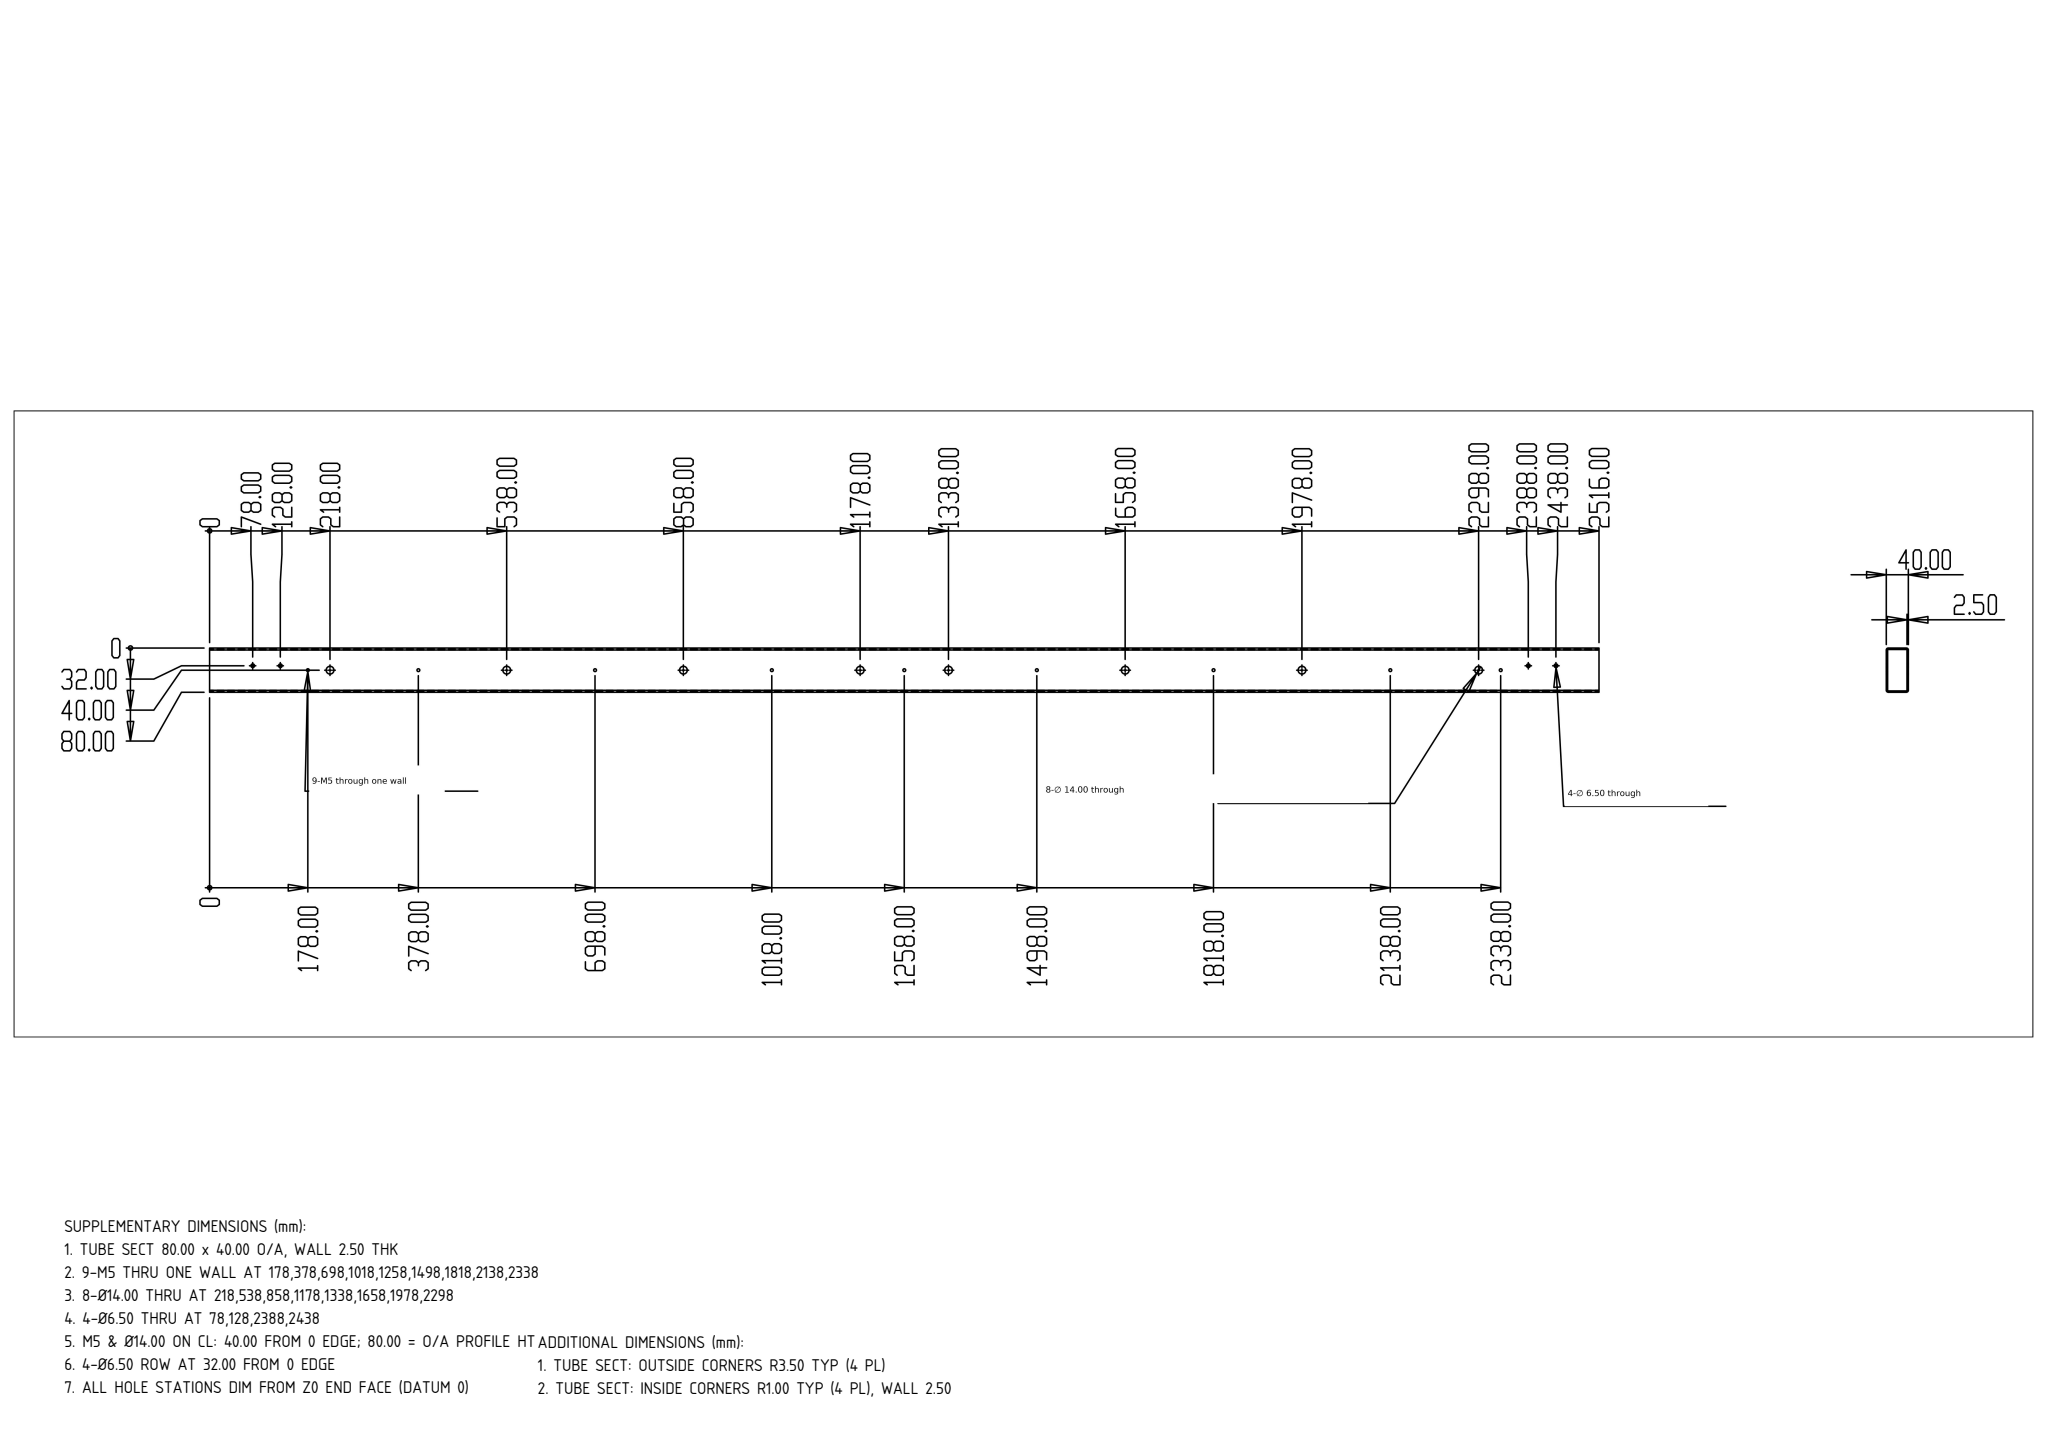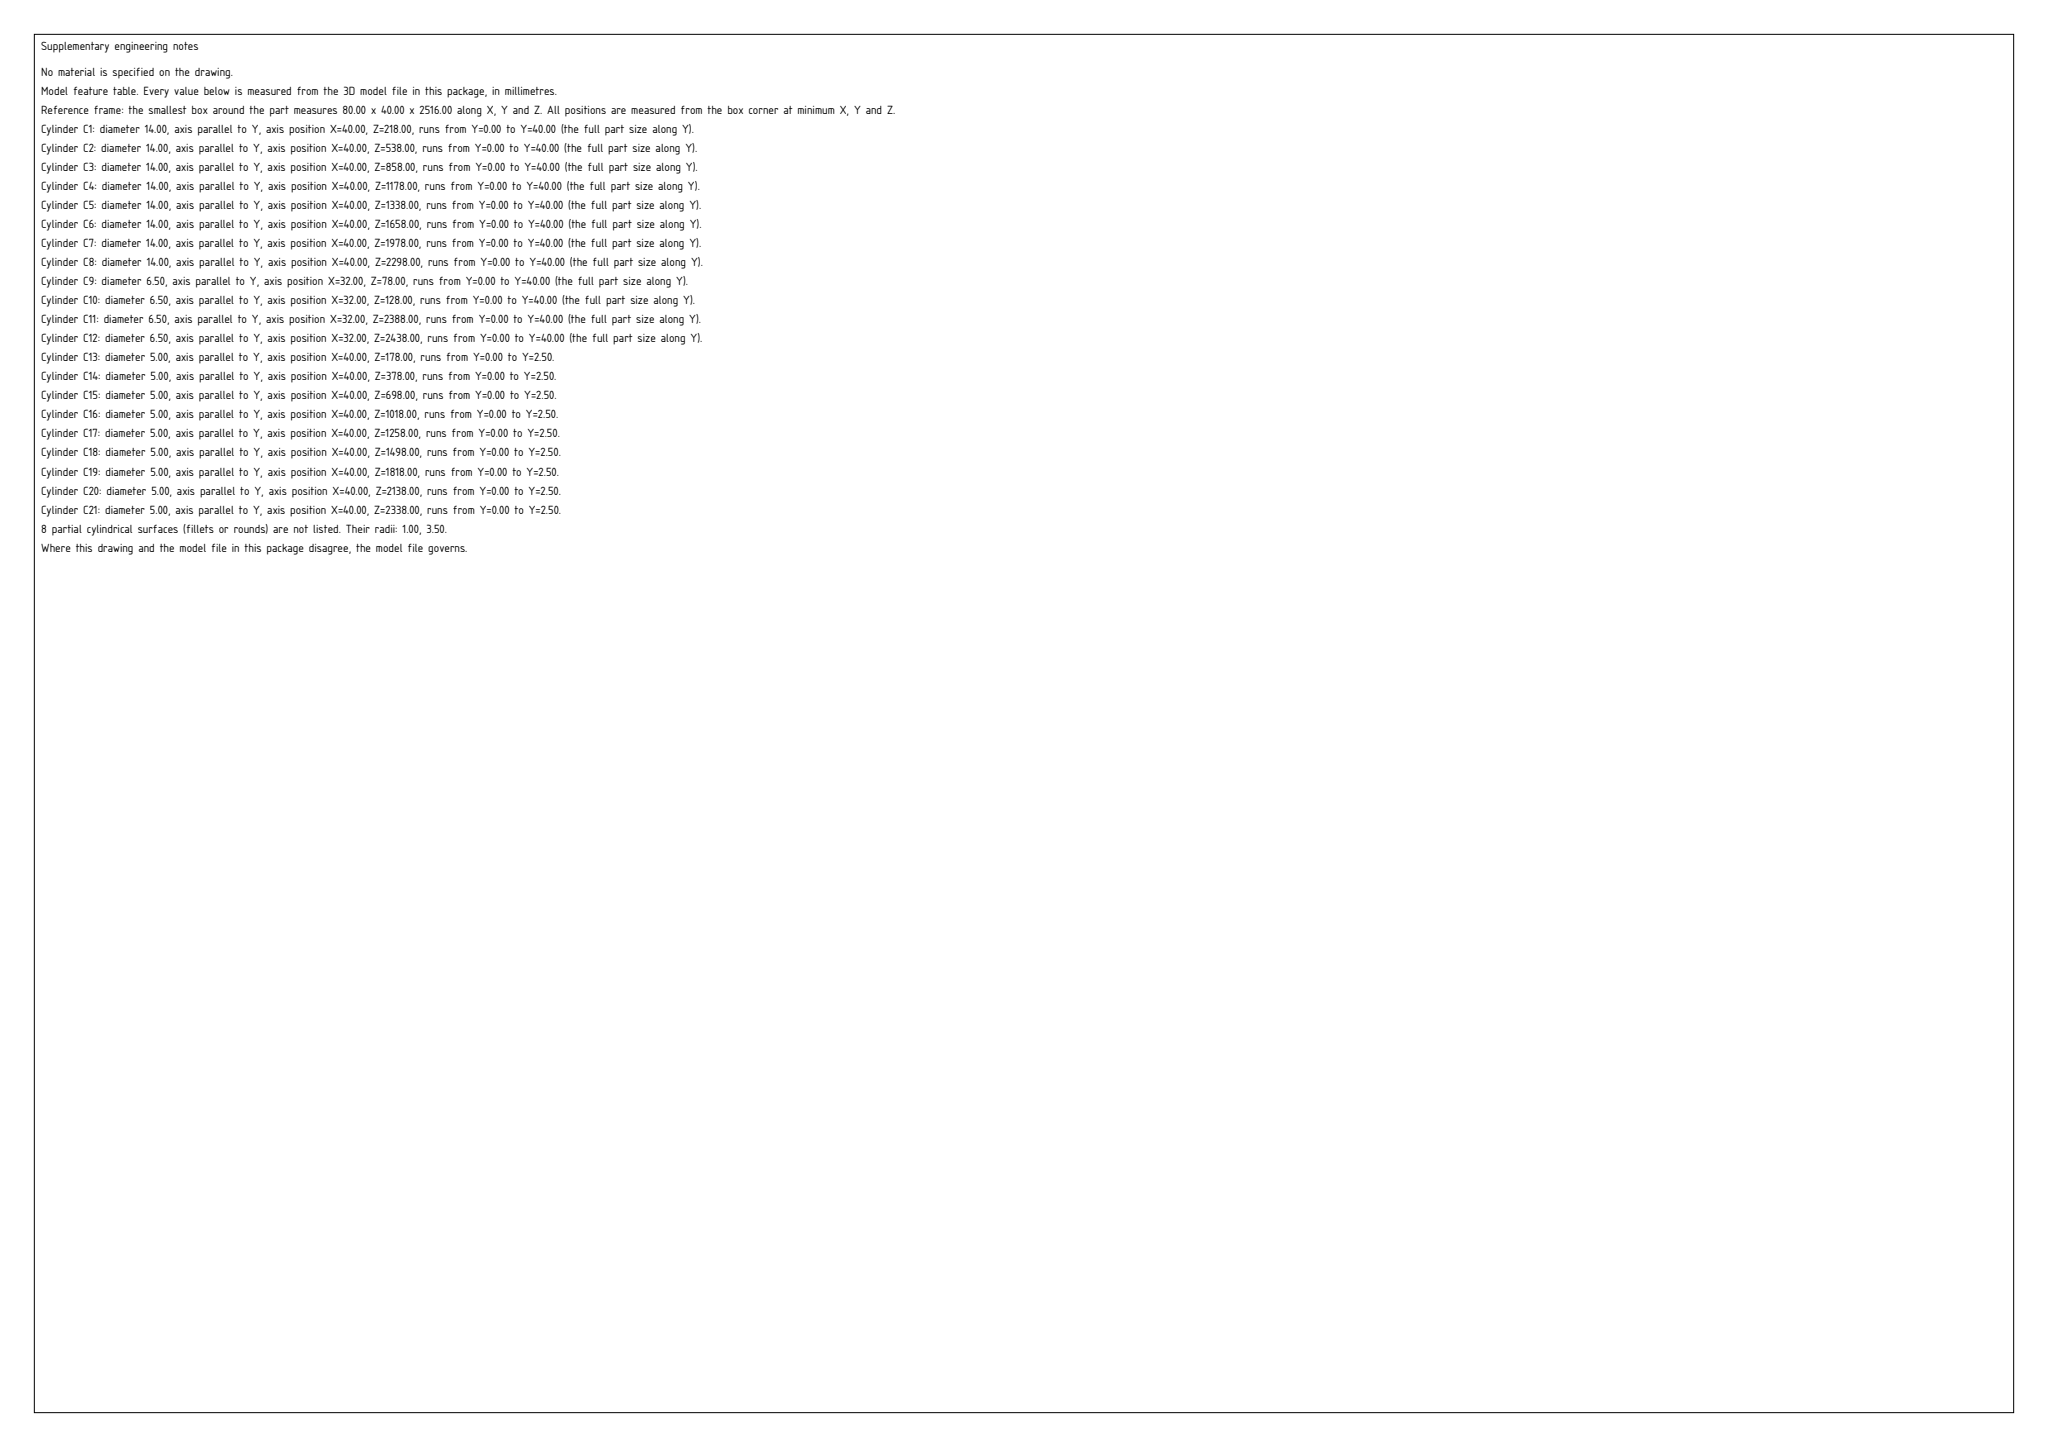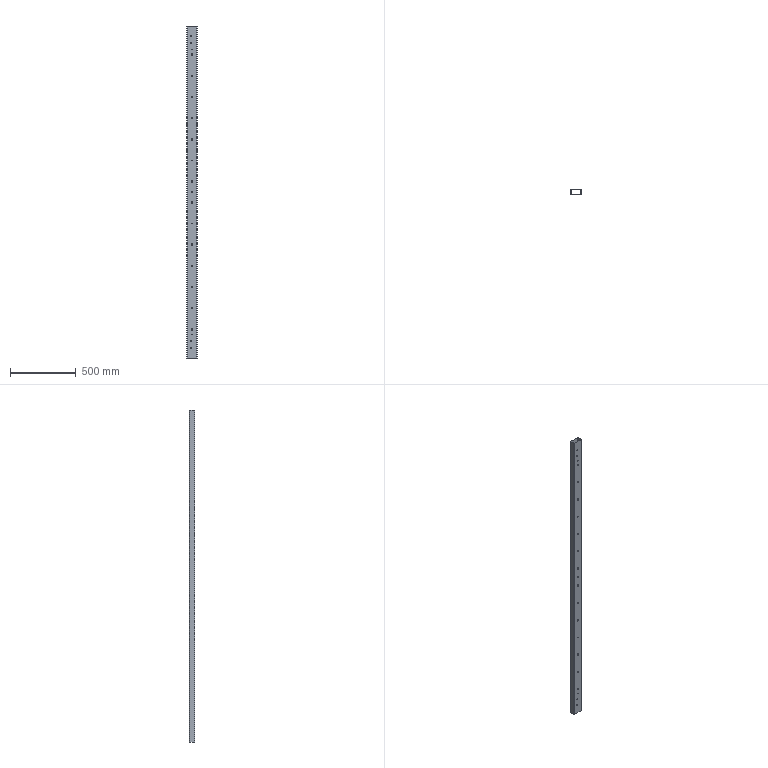Part | SolidWorks | mm | 1 solid | 84 faces | box 80 x 40 x 2516 mm | volume 1415140 mm3 | cylinder 74 | plane 10 | commonest cylinder face diameters 14 x32 5 x18 6.5 x16 7 x4 2 x4
build123d program:
from build123d import *

# Parameters (mm, degrees)
BOSS_EXTRUDE1_DEPTH = 2516
CUT_EXTRUDE1_REACH  = 2518.636
CUT_EXTRUDE2_START  = -37.5
CUT_EXTRUDE2_DEPTH  = 37.5


with BuildPart() as part:
    # Sketch1 → Boss-Extrude1 (new body)
    with BuildSketch(Plane.XY):
        with BuildLine():
            Line((40, -16.5), (40, 16.5))
            ThreePointArc((40, 16.5), (38.975, 18.975), (36.5, 20))
            Line((36.5, 20), (-36.5, 20))
            ThreePointArc((-36.5, 20), (-38.975, 18.975), (-40, 16.5))
            Line((-40, 16.5), (-40, -16.5))
            ThreePointArc((-40, -16.5), (-38.975, -18.975), (-36.5, -20))
            Line((-36.5, -20), (36.5, -20))
            ThreePointArc((36.5, -20), (38.975, -18.975), (40, -16.5))
        make_face()
        with BuildLine():
            Line((37.5, -16.5), (37.5, 16.5))
            ThreePointArc((37.5, 16.5), (37.207, 17.207), (36.5, 17.5))
            Line((36.5, 17.5), (-36.5, 17.5))
            ThreePointArc((-36.5, 17.5), (-37.207, 17.207), (-37.5, 16.5))
            Line((-37.5, 16.5), (-37.5, -16.5))
            ThreePointArc((-37.5, -16.5), (-37.207, -17.207), (-36.5, -17.5))
            Line((-36.5, -17.5), (36.5, -17.5))
            ThreePointArc((36.5, -17.5), (37.207, -17.207), (37.5, -16.5))
        make_face(mode=Mode.SUBTRACT)
    extrude(amount=BOSS_EXTRUDE1_DEPTH)

    # Cut-Extrude1: up to this face of the body (flat: up to its plane)
    cut_extrude1_end = Plane(part.part.faces().sort_by_distance((0, -20, 1258))[0])
    # Sketch2 → Cut-Extrude1 (cut, up to the picked face)
    with BuildSketch(Plane(origin=(0, 20, 0), x_dir=(1, 0, 0), z_dir=(0, 1, 0)), mode=Mode.PRIVATE) as cut_extrude1_sk1:
        with BuildLine():
            ThreePointArc((7, -2298), (0, -2291), (-7, -2298))
            ThreePointArc((-7, -2298), (0, -2305), (7, -2298))
        make_face()
    cut_extrude1_tool1 = split(extrude(cut_extrude1_sk1.sketch, amount=-CUT_EXTRUDE1_REACH, mode=Mode.PRIVATE), bisect_by=cut_extrude1_end, keep=Keep.BOTH, mode=Mode.PRIVATE)
    # Sketch2 → Cut-Extrude1 (cut, up to the picked face)
    with BuildSketch(Plane(origin=(0, 20, 0), x_dir=(1, 0, 0), z_dir=(0, 1, 0)), mode=Mode.PRIVATE) as cut_extrude1_sk2:
        with BuildLine():
            ThreePointArc((7, -218), (0, -211), (-7, -218))
            ThreePointArc((-7, -218), (0, -225), (7, -218))
        make_face()
    cut_extrude1_tool2 = split(extrude(cut_extrude1_sk2.sketch, amount=-CUT_EXTRUDE1_REACH, mode=Mode.PRIVATE), bisect_by=cut_extrude1_end, keep=Keep.BOTH, mode=Mode.PRIVATE)
    # Sketch2 → Cut-Extrude1 (cut, up to the picked face)
    with BuildSketch(Plane(origin=(0, 20, 0), x_dir=(1, 0, 0), z_dir=(0, 1, 0)), mode=Mode.PRIVATE) as cut_extrude1_sk3:
        with BuildLine():
            ThreePointArc((7, -1658), (0, -1651), (-7, -1658))
            ThreePointArc((-7, -1658), (0, -1665), (7, -1658))
        make_face()
    cut_extrude1_tool3 = split(extrude(cut_extrude1_sk3.sketch, amount=-CUT_EXTRUDE1_REACH, mode=Mode.PRIVATE), bisect_by=cut_extrude1_end, keep=Keep.BOTH, mode=Mode.PRIVATE)
    # Sketch2 → Cut-Extrude1 (cut, up to the picked face)
    with BuildSketch(Plane(origin=(0, 20, 0), x_dir=(1, 0, 0), z_dir=(0, 1, 0)), mode=Mode.PRIVATE) as cut_extrude1_sk4:
        with BuildLine():
            ThreePointArc((7, -1978), (0, -1971), (-7, -1978))
            ThreePointArc((-7, -1978), (0, -1985), (7, -1978))
        make_face()
    cut_extrude1_tool4 = split(extrude(cut_extrude1_sk4.sketch, amount=-CUT_EXTRUDE1_REACH, mode=Mode.PRIVATE), bisect_by=cut_extrude1_end, keep=Keep.BOTH, mode=Mode.PRIVATE)
    # Sketch2 → Cut-Extrude1 (cut, up to the picked face)
    with BuildSketch(Plane(origin=(0, 20, 0), x_dir=(1, 0, 0), z_dir=(0, 1, 0)), mode=Mode.PRIVATE) as cut_extrude1_sk5:
        with BuildLine():
            ThreePointArc((7, -538), (0, -531), (-7, -538))
            ThreePointArc((-7, -538), (0, -545), (7, -538))
        make_face()
    cut_extrude1_tool5 = split(extrude(cut_extrude1_sk5.sketch, amount=-CUT_EXTRUDE1_REACH, mode=Mode.PRIVATE), bisect_by=cut_extrude1_end, keep=Keep.BOTH, mode=Mode.PRIVATE)
    # Sketch2 → Cut-Extrude1 (cut, up to the picked face)
    with BuildSketch(Plane(origin=(0, 20, 0), x_dir=(1, 0, 0), z_dir=(0, 1, 0)), mode=Mode.PRIVATE) as cut_extrude1_sk6:
        with BuildLine():
            ThreePointArc((7, -858), (0, -851), (-7, -858))
            ThreePointArc((-7, -858), (0, -865), (7, -858))
        make_face()
    cut_extrude1_tool6 = split(extrude(cut_extrude1_sk6.sketch, amount=-CUT_EXTRUDE1_REACH, mode=Mode.PRIVATE), bisect_by=cut_extrude1_end, keep=Keep.BOTH, mode=Mode.PRIVATE)
    # Sketch2 → Cut-Extrude1 (cut, up to the picked face)
    with BuildSketch(Plane(origin=(0, 20, 0), x_dir=(1, 0, 0), z_dir=(0, 1, 0)), mode=Mode.PRIVATE) as cut_extrude1_sk7:
        with BuildLine():
            ThreePointArc((7, -1178), (0, -1171), (-7, -1178))
            ThreePointArc((-7, -1178), (0, -1185), (7, -1178))
        make_face()
    cut_extrude1_tool7 = split(extrude(cut_extrude1_sk7.sketch, amount=-CUT_EXTRUDE1_REACH, mode=Mode.PRIVATE), bisect_by=cut_extrude1_end, keep=Keep.BOTH, mode=Mode.PRIVATE)
    # Sketch2 → Cut-Extrude1 (cut, up to the picked face)
    with BuildSketch(Plane(origin=(0, 20, 0), x_dir=(1, 0, 0), z_dir=(0, 1, 0)), mode=Mode.PRIVATE) as cut_extrude1_sk8:
        with BuildLine():
            ThreePointArc((7, -1338), (0, -1331), (-7, -1338))
            ThreePointArc((-7, -1338), (0, -1345), (7, -1338))
        make_face()
    cut_extrude1_tool8 = split(extrude(cut_extrude1_sk8.sketch, amount=-CUT_EXTRUDE1_REACH, mode=Mode.PRIVATE), bisect_by=cut_extrude1_end, keep=Keep.BOTH, mode=Mode.PRIVATE)
    # Sketch2 → Cut-Extrude1 (cut, up to the picked face)
    with BuildSketch(Plane(origin=(0, 20, 0), x_dir=(1, 0, 0), z_dir=(0, 1, 0)), mode=Mode.PRIVATE) as cut_extrude1_sk9:
        with BuildLine():
            ThreePointArc((-8, -74.75), (-11.25, -78), (-8, -81.25))
            ThreePointArc((-8, -81.25), (-4.75, -78), (-8, -74.75))
        make_face()
    cut_extrude1_tool9 = split(extrude(cut_extrude1_sk9.sketch, amount=-CUT_EXTRUDE1_REACH, mode=Mode.PRIVATE), bisect_by=cut_extrude1_end, keep=Keep.BOTH, mode=Mode.PRIVATE)
    # Sketch2 → Cut-Extrude1 (cut, up to the picked face)
    with BuildSketch(Plane(origin=(0, 20, 0), x_dir=(1, 0, 0), z_dir=(0, 1, 0)), mode=Mode.PRIVATE) as cut_extrude1_sk10:
        with BuildLine():
            ThreePointArc((-8, -124.75), (-11.25, -128), (-8, -131.25))
            ThreePointArc((-8, -131.25), (-4.75, -128), (-8, -124.75))
        make_face()
    cut_extrude1_tool10 = split(extrude(cut_extrude1_sk10.sketch, amount=-CUT_EXTRUDE1_REACH, mode=Mode.PRIVATE), bisect_by=cut_extrude1_end, keep=Keep.BOTH, mode=Mode.PRIVATE)
    # Sketch2 → Cut-Extrude1 (cut, up to the picked face)
    with BuildSketch(Plane(origin=(0, 20, 0), x_dir=(1, 0, 0), z_dir=(0, 1, 0)), mode=Mode.PRIVATE) as cut_extrude1_sk11:
        with BuildLine():
            ThreePointArc((-8, -2384.75), (-11.25, -2388), (-8, -2391.25))
            ThreePointArc((-8, -2391.25), (-4.75, -2388), (-8, -2384.75))
        make_face()
    cut_extrude1_tool11 = split(extrude(cut_extrude1_sk11.sketch, amount=-CUT_EXTRUDE1_REACH, mode=Mode.PRIVATE), bisect_by=cut_extrude1_end, keep=Keep.BOTH, mode=Mode.PRIVATE)
    # Sketch2 → Cut-Extrude1 (cut, up to the picked face)
    with BuildSketch(Plane(origin=(0, 20, 0), x_dir=(1, 0, 0), z_dir=(0, 1, 0)), mode=Mode.PRIVATE) as cut_extrude1_sk12:
        with BuildLine():
            ThreePointArc((-8, -2434.75), (-11.25, -2438), (-8, -2441.25))
            ThreePointArc((-8, -2441.25), (-4.75, -2438), (-8, -2434.75))
        make_face()
    cut_extrude1_tool12 = split(extrude(cut_extrude1_sk12.sketch, amount=-CUT_EXTRUDE1_REACH, mode=Mode.PRIVATE), bisect_by=cut_extrude1_end, keep=Keep.BOTH, mode=Mode.PRIVATE)
    add(cut_extrude1_tool1.solids().sort_by(Axis((0, 20, 2298), (0, -1, 0)))[0], mode=Mode.SUBTRACT)
    add(cut_extrude1_tool2.solids().sort_by(Axis((0, 20, 218), (0, -1, 0)))[0], mode=Mode.SUBTRACT)
    add(cut_extrude1_tool3.solids().sort_by(Axis((0, 20, 1658), (0, -1, 0)))[0], mode=Mode.SUBTRACT)
    add(cut_extrude1_tool4.solids().sort_by(Axis((0, 20, 1978), (0, -1, 0)))[0], mode=Mode.SUBTRACT)
    add(cut_extrude1_tool5.solids().sort_by(Axis((0, 20, 538), (0, -1, 0)))[0], mode=Mode.SUBTRACT)
    add(cut_extrude1_tool6.solids().sort_by(Axis((0, 20, 858), (0, -1, 0)))[0], mode=Mode.SUBTRACT)
    add(cut_extrude1_tool7.solids().sort_by(Axis((0, 20, 1178), (0, -1, 0)))[0], mode=Mode.SUBTRACT)
    add(cut_extrude1_tool8.solids().sort_by(Axis((0, 20, 1338), (0, -1, 0)))[0], mode=Mode.SUBTRACT)
    add(cut_extrude1_tool9.solids().sort_by(Axis((-8, 20, 78), (0, -1, 0)))[0], mode=Mode.SUBTRACT)
    add(cut_extrude1_tool10.solids().sort_by(Axis((-8, 20, 128), (0, -1, 0)))[0], mode=Mode.SUBTRACT)
    add(cut_extrude1_tool11.solids().sort_by(Axis((-8, 20, 2388), (0, -1, 0)))[0], mode=Mode.SUBTRACT)
    add(cut_extrude1_tool12.solids().sort_by(Axis((-8, 20, 2438), (0, -1, 0)))[0], mode=Mode.SUBTRACT)

    # Sketch3 → Cut-Extrude2 (cut)
    with BuildSketch(Plane.XZ.offset(20).offset(CUT_EXTRUDE2_START)):
        with BuildLine():
            ThreePointArc((-7, 1178), (0, 1171), (7, 1178))
            ThreePointArc((7, 1178), (0, 1185), (-7, 1178))
        make_face()
        with BuildLine():
            ThreePointArc((-8, 81.25), (-11.25, 78), (-8, 74.75))
            ThreePointArc((-8, 74.75), (-4.75, 78), (-8, 81.25))
        make_face()
        with BuildLine():
            ThreePointArc((-8, 131.25), (-11.25, 128), (-8, 124.75))
            ThreePointArc((-8, 124.75), (-4.75, 128), (-8, 131.25))
        make_face()
        with BuildLine():
            ThreePointArc((-8, 2391.25), (-11.25, 2388), (-8, 2384.75))
            ThreePointArc((-8, 2384.75), (-4.75, 2388), (-8, 2391.25))
        make_face()
        with BuildLine():
            ThreePointArc((-8, 2441.25), (-11.25, 2438), (-8, 2434.75))
            ThreePointArc((-8, 2434.75), (-4.75, 2438), (-8, 2441.25))
        make_face()
        with BuildLine():
            ThreePointArc((0, 2335.5), (2.5, 2338), (0, 2340.5))
            ThreePointArc((0, 2340.5), (-2.5, 2338), (0, 2335.5))
        make_face()
        with BuildLine():
            ThreePointArc((0, 2135.5), (2.5, 2138), (0, 2140.5))
            ThreePointArc((0, 2140.5), (-2.5, 2138), (0, 2135.5))
        make_face()
        with BuildLine():
            ThreePointArc((0, 1815.5), (2.5, 1818), (0, 1820.5))
            ThreePointArc((0, 1820.5), (-2.5, 1818), (0, 1815.5))
        make_face()
        with BuildLine():
            ThreePointArc((0, 1495.5), (2.5, 1498), (0, 1500.5))
            ThreePointArc((0, 1500.5), (-2.5, 1498), (0, 1495.5))
        make_face()
        with BuildLine():
            ThreePointArc((0, 1255.5), (2.5, 1258), (0, 1260.5))
            ThreePointArc((0, 1260.5), (-2.5, 1258), (0, 1255.5))
        make_face()
        with BuildLine():
            ThreePointArc((0, 1015.5), (2.5, 1018), (0, 1020.5))
            ThreePointArc((0, 1020.5), (-2.5, 1018), (0, 1015.5))
        make_face()
        with BuildLine():
            ThreePointArc((0, 695.5), (2.5, 698), (0, 700.5))
            ThreePointArc((0, 700.5), (-2.5, 698), (0, 695.5))
        make_face()
        with BuildLine():
            ThreePointArc((0, 375.5), (2.5, 378), (0, 380.5))
            ThreePointArc((0, 380.5), (-2.5, 378), (0, 375.5))
        make_face()
        with BuildLine():
            ThreePointArc((0, 175.5), (2.5, 178), (0, 180.5))
            ThreePointArc((0, 180.5), (-2.5, 178), (0, 175.5))
        make_face()
        with BuildLine():
            ThreePointArc((-7, 1338), (0, 1331), (7, 1338))
            ThreePointArc((7, 1338), (0, 1345), (-7, 1338))
        make_face()
        with BuildLine():
            ThreePointArc((-7, 218), (0, 211), (7, 218))
            ThreePointArc((7, 218), (0, 225), (-7, 218))
        make_face()
        with BuildLine():
            ThreePointArc((-7, 1978), (0, 1971), (7, 1978))
            ThreePointArc((7, 1978), (0, 1985), (-7, 1978))
        make_face()
        with BuildLine():
            ThreePointArc((-7, 2298), (0, 2291), (7, 2298))
            ThreePointArc((7, 2298), (0, 2305), (-7, 2298))
        make_face()
        with BuildLine():
            ThreePointArc((-7, 858), (0, 851), (7, 858))
            ThreePointArc((7, 858), (0, 865), (-7, 858))
        make_face()
        with BuildLine():
            ThreePointArc((-7, 538), (0, 531), (7, 538))
            ThreePointArc((7, 538), (0, 545), (-7, 538))
        make_face()
        with BuildLine():
            ThreePointArc((-7, 1658), (0, 1651), (7, 1658))
            ThreePointArc((7, 1658), (0, 1665), (-7, 1658))
        make_face()
    extrude(amount=CUT_EXTRUDE2_DEPTH, mode=Mode.SUBTRACT)


solid = part.part